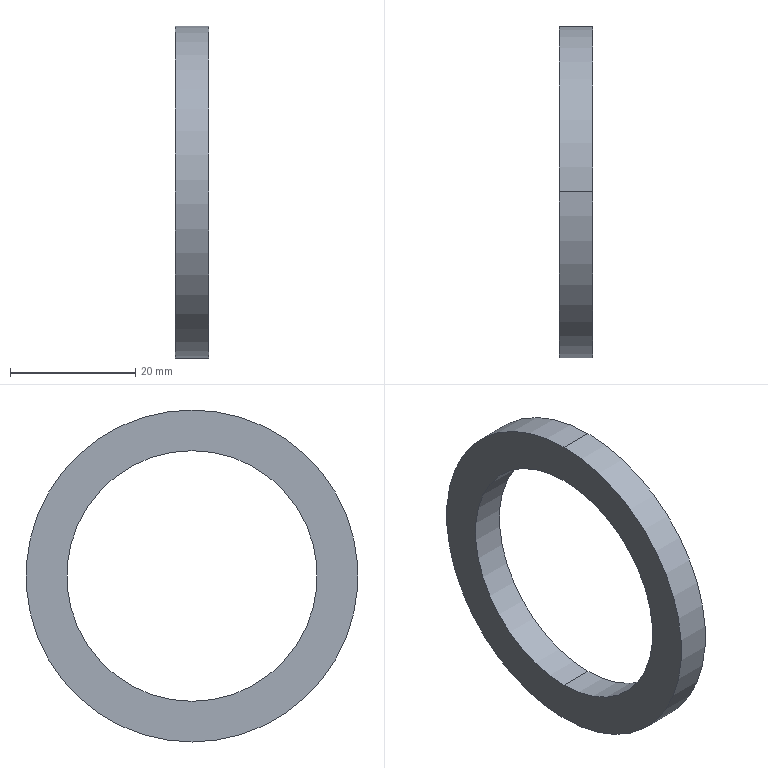Component | SolidWorks | 4OilSeal-1 | 1 solid | 6 faces | box 5.4 x 53 x 53 mm | volume 5128 mm3 | cylinder 4 | plane 2 | commonest cylinder face diameters 40 x2 53 x2
build123d program:
from build123d import *

# Parameters (mm, degrees)
SKETCH44_R           = 26.5
SKETCH44_R_2         = 20
BOSS_EXTRUDE10_DEPTH = 5.4


with BuildPart() as part:
    # Sketch44 → Boss-Extrude10 (new body)
    with BuildSketch(Plane(origin=(0, 0, 0), x_dir=(1, 0, 0), z_dir=(0, 1, 0))):
        with Locations(Location((0, 0, 0), (0, 0, 90))):
            Circle(SKETCH44_R)
        with Locations(Location((0, 0, 0), (0, 0, 90))):
            Circle(SKETCH44_R_2, mode=Mode.SUBTRACT)
    extrude(amount=BOSS_EXTRUDE10_DEPTH)


solid = part.part

# Placed as in the assembly
solid = solid.moved(Location((-156.715, -90.191, 512), (0, 0, 90)))
STEP:
#1=CARTESIAN_POINT('',(-6.17,-3.551,19.37));
#2=VERTEX_POINT('',#1);
#3=CARTESIAN_POINT('',(-6.17,-3.551,20.945));
#4=VERTEX_POINT('',#3);
#5=CARTESIAN_POINT('',(-6.17,-3.551,20.157));
#6=DIRECTION('',(1.,0.,0.));
#7=DIRECTION('',(0.,0.,1.));
#8=AXIS2_PLACEMENT_3D('',#5,#6,#7);
#9=CIRCLE('',#8,0.7874);
#10=EDGE_CURVE('',#2,#4,#9,.T.);
#11=ORIENTED_EDGE('',*,*,#10,.T.);
#12=CARTESIAN_POINT('',(-6.382,-3.551,20.945));
#13=VERTEX_POINT('',#12);
#14=CARTESIAN_POINT('',(-6.17,-3.551,20.945));
#15=DIRECTION('',(-1.,0.,0.));
#16=VECTOR('',#15,39.37);
#17=LINE('',#14,#16);
#18=EDGE_CURVE('',#4,#13,#17,.T.);
#19=ORIENTED_EDGE('',*,*,#18,.T.);
#20=CARTESIAN_POINT('',(-6.382,-3.551,19.37));
#21=VERTEX_POINT('',#20);
#22=CARTESIAN_POINT('',(-6.382,-3.551,20.157));
#23=DIRECTION('',(1.,0.,0.));
#24=DIRECTION('',(0.,0.,1.));
#25=AXIS2_PLACEMENT_3D('',#22,#23,#24);
#26=CIRCLE('',#25,0.7874);
#27=EDGE_CURVE('',#21,#13,#26,.T.);
#28=ORIENTED_EDGE('',*,*,#27,.F.);
#29=CARTESIAN_POINT('',(-6.17,-3.551,19.37));
#30=DIRECTION('',(-1.,0.,0.));
#31=VECTOR('',#30,39.37);
#32=LINE('',#29,#31);
#33=EDGE_CURVE('',#2,#21,#32,.T.);
#34=ORIENTED_EDGE('',*,*,#33,.F.);
#35=EDGE_LOOP('',(#11,#19,#28,#34));
#36=FACE_OUTER_BOUND('',#35,.T.);
#37=CARTESIAN_POINT('',(-6.17,-3.551,20.157));
#38=DIRECTION('',(-1.,0.,0.));
#39=DIRECTION('',(0.,0.,-1.));
#40=AXIS2_PLACEMENT_3D('',#37,#38,#39);
#41=CYLINDRICAL_SURFACE('',#40,0.7874);
#42=ADVANCED_FACE('',(#36),#41,.F.);
#43=CARTESIAN_POINT('',(-6.17,-3.551,21.201));
#44=VERTEX_POINT('',#43);
#45=CARTESIAN_POINT('',(-6.17,-3.551,19.114));
#46=VERTEX_POINT('',#45);
#47=CARTESIAN_POINT('',(-6.17,-3.551,20.157));
#48=DIRECTION('',(1.,0.,0.));
#49=DIRECTION('',(0.,0.,1.));
#50=AXIS2_PLACEMENT_3D('',#47,#48,#49);
#51=CIRCLE('',#50,1.043);
#52=EDGE_CURVE('',#44,#46,#51,.T.);
#53=ORIENTED_EDGE('',*,*,#52,.F.);
#54=CARTESIAN_POINT('',(-6.382,-3.551,21.201));
#55=VERTEX_POINT('',#54);
#56=CARTESIAN_POINT('',(-6.17,-3.551,21.201));
#57=DIRECTION('',(-1.,0.,0.));
#58=VECTOR('',#57,39.37);
#59=LINE('',#56,#58);
#60=EDGE_CURVE('',#44,#55,#59,.T.);
#61=ORIENTED_EDGE('',*,*,#60,.T.);
#62=CARTESIAN_POINT('',(-6.382,-3.551,19.114));
#63=VERTEX_POINT('',#62);
#64=CARTESIAN_POINT('',(-6.382,-3.551,20.157));
#65=DIRECTION('',(1.,0.,0.));
#66=DIRECTION('',(0.,0.,1.));
#67=AXIS2_PLACEMENT_3D('',#64,#65,#66);
#68=CIRCLE('',#67,1.043);
#69=EDGE_CURVE('',#55,#63,#68,.T.);
#70=ORIENTED_EDGE('',*,*,#69,.T.);
#71=CARTESIAN_POINT('',(-6.17,-3.551,19.114));
#72=DIRECTION('',(-1.,0.,0.));
#73=VECTOR('',#72,39.37);
#74=LINE('',#71,#73);
#75=EDGE_CURVE('',#46,#63,#74,.T.);
#76=ORIENTED_EDGE('',*,*,#75,.F.);
#77=EDGE_LOOP('',(#53,#61,#70,#76));
#78=FACE_OUTER_BOUND('',#77,.T.);
#79=CARTESIAN_POINT('',(-6.17,-3.551,20.157));
#80=DIRECTION('',(-1.,0.,0.));
#81=DIRECTION('',(0.,0.,-1.));
#82=AXIS2_PLACEMENT_3D('',#79,#80,#81);
#83=CYLINDRICAL_SURFACE('',#82,1.043);
#84=ADVANCED_FACE('',(#78),#83,.T.);
#85=CARTESIAN_POINT('',(-6.17,-3.551,20.157));
#86=DIRECTION('',(1.,0.,0.));
#87=DIRECTION('',(0.,0.,1.));
#88=AXIS2_PLACEMENT_3D('',#85,#86,#87);
#89=CIRCLE('',#88,1.043);
#90=EDGE_CURVE('',#46,#44,#89,.T.);
#91=ORIENTED_EDGE('',*,*,#90,.T.);
#92=ORIENTED_EDGE('',*,*,#52,.T.);
#93=EDGE_LOOP('',(#91,#92));
#94=FACE_OUTER_BOUND('',#93,.T.);
#95=ORIENTED_EDGE('',*,*,#10,.F.);
#96=CARTESIAN_POINT('',(-6.17,-3.551,20.157));
#97=DIRECTION('',(1.,0.,0.));
#98=DIRECTION('',(0.,0.,1.));
#99=AXIS2_PLACEMENT_3D('',#96,#97,#98);
#100=CIRCLE('',#99,0.7874);
#101=EDGE_CURVE('',#4,#2,#100,.T.);
#102=ORIENTED_EDGE('',*,*,#101,.F.);
#103=EDGE_LOOP('',(#95,#102));
#104=FACE_BOUND('',#103,.T.);
#105=CARTESIAN_POINT('',(-6.17,-3.551,20.157));
#106=DIRECTION('',(1.,0.,0.));
#107=DIRECTION('',(0.,0.,1.));
#108=AXIS2_PLACEMENT_3D('',#105,#106,#107);
#109=PLANE('',#108);
#110=ADVANCED_FACE('',(#94,#104),#109,.T.);
#111=CARTESIAN_POINT('',(-6.382,-3.551,20.157));
#112=DIRECTION('',(1.,0.,0.));
#113=DIRECTION('',(0.,0.,1.));
#114=AXIS2_PLACEMENT_3D('',#111,#112,#113);
#115=CIRCLE('',#114,1.043);
#116=EDGE_CURVE('',#63,#55,#115,.T.);
#117=ORIENTED_EDGE('',*,*,#116,.F.);
#118=ORIENTED_EDGE('',*,*,#69,.F.);
#119=EDGE_LOOP('',(#117,#118));
#120=FACE_OUTER_BOUND('',#119,.T.);
#121=ORIENTED_EDGE('',*,*,#27,.T.);
#122=CARTESIAN_POINT('',(-6.382,-3.551,20.157));
#123=DIRECTION('',(1.,0.,0.));
#124=DIRECTION('',(0.,0.,1.));
#125=AXIS2_PLACEMENT_3D('',#122,#123,#124);
#126=CIRCLE('',#125,0.7874);
#127=EDGE_CURVE('',#13,#21,#126,.T.);
#128=ORIENTED_EDGE('',*,*,#127,.T.);
#129=EDGE_LOOP('',(#121,#128));
#130=FACE_BOUND('',#129,.T.);
#131=CARTESIAN_POINT('',(-6.382,-3.551,20.157));
#132=DIRECTION('',(1.,0.,0.));
#133=DIRECTION('',(0.,0.,1.));
#134=AXIS2_PLACEMENT_3D('',#131,#132,#133);
#135=PLANE('',#134);
#136=ADVANCED_FACE('',(#120,#130),#135,.F.);
#137=ORIENTED_EDGE('',*,*,#60,.F.);
#138=ORIENTED_EDGE('',*,*,#90,.F.);
#139=ORIENTED_EDGE('',*,*,#75,.T.);
#140=ORIENTED_EDGE('',*,*,#116,.T.);
#141=EDGE_LOOP('',(#137,#138,#139,#140));
#142=FACE_OUTER_BOUND('',#141,.T.);
#143=CARTESIAN_POINT('',(-6.17,-3.551,20.157));
#144=DIRECTION('',(-1.,0.,0.));
#145=DIRECTION('',(0.,0.,-1.));
#146=AXIS2_PLACEMENT_3D('',#143,#144,#145);
#147=CYLINDRICAL_SURFACE('',#146,1.043);
#148=ADVANCED_FACE('',(#142),#147,.T.);
#149=ORIENTED_EDGE('',*,*,#18,.F.);
#150=ORIENTED_EDGE('',*,*,#101,.T.);
#151=ORIENTED_EDGE('',*,*,#33,.T.);
#152=ORIENTED_EDGE('',*,*,#127,.F.);
#153=EDGE_LOOP('',(#149,#150,#151,#152));
#154=FACE_OUTER_BOUND('',#153,.T.);
#155=CARTESIAN_POINT('',(-6.17,-3.551,20.157));
#156=DIRECTION('',(-1.,0.,0.));
#157=DIRECTION('',(0.,0.,-1.));
#158=AXIS2_PLACEMENT_3D('',#155,#156,#157);
#159=CYLINDRICAL_SURFACE('',#158,0.7874);
#160=ADVANCED_FACE('',(#154),#159,.F.);
#161=CLOSED_SHELL('',(#42,#84,#110,#136,#148,#160));
#162=MANIFOLD_SOLID_BREP('',#161);
#163=CARTESIAN_POINT('',(0.,0.,0.));
#164=DIRECTION('',(0.,0.,1.));
#165=DIRECTION('',(1.,0.,0.));
#166=AXIS2_PLACEMENT_3D('',#163,#164,#165);
#167=(LENGTH_UNIT()NAMED_UNIT(*)SI_UNIT($,.METRE.));
#168=LENGTH_MEASURE_WITH_UNIT(LENGTH_MEASURE(0.0254),#167);
#169=DIMENSIONAL_EXPONENTS(1.,0.,0.,0.,0.,0.,0.);
#170=(CONVERSION_BASED_UNIT('',#168)LENGTH_UNIT()NAMED_UNIT(#169));
#171=UNCERTAINTY_MEASURE_WITH_UNIT(LENGTH_MEASURE(0.00001),#170,'','');
#172=(NAMED_UNIT(*)PLANE_ANGLE_UNIT()SI_UNIT($,.RADIAN.));
#173=(NAMED_UNIT(*)SI_UNIT($,.STERADIAN.)SOLID_ANGLE_UNIT());
#174=(GEOMETRIC_REPRESENTATION_CONTEXT(3)GLOBAL_UNCERTAINTY_ASSIGNED_CONTEXT((#171))GLOBAL_UNIT_ASSIGNED_CONTEXT((#170,#172,#173))REPRESENTATION_CONTEXT('',''));
#175=ADVANCED_BREP_SHAPE_REPRESENTATION('',(#162,#166),#174);
#176=COLOUR_RGB('',0.7922,0.8196,0.9333);
#177=FILL_AREA_STYLE_COLOUR('',#176);
#178=FILL_AREA_STYLE('',(#177));
#179=SURFACE_STYLE_FILL_AREA(#178);
#180=SURFACE_SIDE_STYLE('',(#179));
#181=SURFACE_STYLE_USAGE(.BOTH.,#180);
#182=PRESENTATION_STYLE_ASSIGNMENT((#181));
#183=STYLED_ITEM('',(#182),#162);
#184=(LENGTH_UNIT()NAMED_UNIT(*)SI_UNIT($,.METRE.));
#185=LENGTH_MEASURE_WITH_UNIT(LENGTH_MEASURE(0.0254),#184);
#186=DIMENSIONAL_EXPONENTS(1.,0.,0.,0.,0.,0.,0.);
#187=(CONVERSION_BASED_UNIT('',#185)LENGTH_UNIT()NAMED_UNIT(#186));
#188=UNCERTAINTY_MEASURE_WITH_UNIT(LENGTH_MEASURE(0.00001),#187,'','');
#189=(NAMED_UNIT(*)PLANE_ANGLE_UNIT()SI_UNIT($,.RADIAN.));
#190=(NAMED_UNIT(*)SI_UNIT($,.STERADIAN.)SOLID_ANGLE_UNIT());
#191=(GEOMETRIC_REPRESENTATION_CONTEXT(3)GLOBAL_UNCERTAINTY_ASSIGNED_CONTEXT((#188))GLOBAL_UNIT_ASSIGNED_CONTEXT((#187,#189,#190))REPRESENTATION_CONTEXT('',''));
#192=MECHANICAL_DESIGN_GEOMETRIC_PRESENTATION_REPRESENTATION('',(#183),#191);
#193=PRESENTATION_LAYER_ASSIGNMENT('','',(#183));